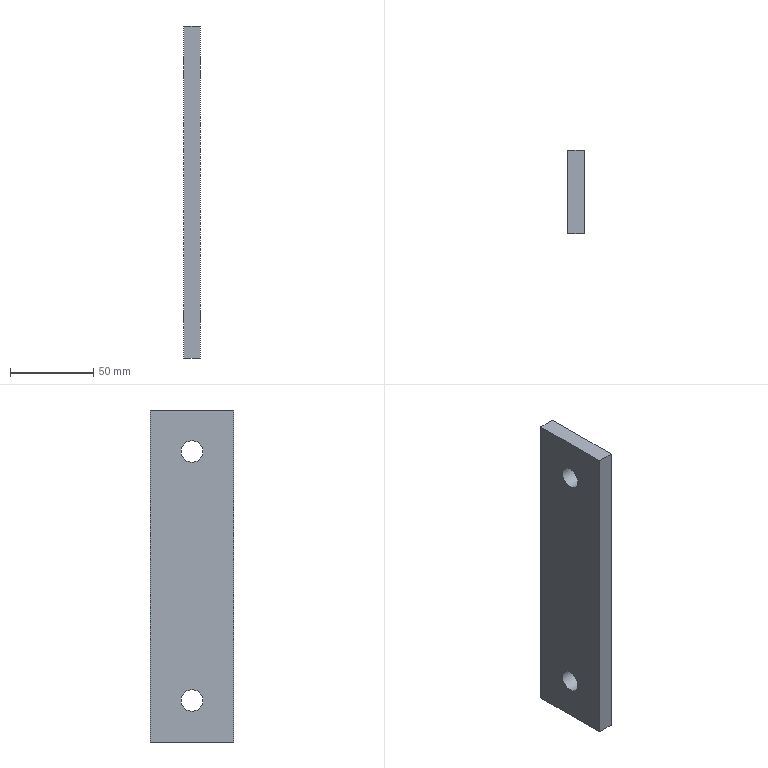Component | NX | BASE_FRAME_SHORT_CONN_PLATE | 1 solid | 8 faces | box 10 x 50 x 200 mm | volume 97345 mm3 | plane 6 | cylinder 2 | commonest cylinder face diameters 13 x2
STEP:
#1=CARTESIAN_POINT('',(0.,0.,0.));
#2=DIRECTION('',(0.,0.,1.));
#3=DIRECTION('',(1.,0.,0.));
#4=AXIS2_PLACEMENT_3D('',#1,#2,#3);
#5=CARTESIAN_POINT('',(-1250.,-50.,100.));
#6=VERTEX_POINT('',#5);
#7=CARTESIAN_POINT('',(-1250.,-50.,-100.));
#8=VERTEX_POINT('',#7);
#9=CARTESIAN_POINT('',(-1250.,-50.,100.));
#10=DIRECTION('',(0.,0.,-1.));
#11=VECTOR('',#10,1.);
#12=LINE('',#9,#11);
#13=CARTESIAN_POINT('',(-1260.,-50.,100.));
#14=DIRECTION('',(0.,-1.,0.));
#15=DIRECTION('',(1.,0.,0.));
#16=AXIS2_PLACEMENT_3D('',#13,#14,#15);
#17=PLANE('',#16);
#18=CARTESIAN_POINT('',(10.,0.));
#19=DIRECTION('',(0.,-1.));
#20=VECTOR('',#19,1.);
#21=LINE('',#18,#20);
#22=(GEOMETRIC_REPRESENTATION_CONTEXT(2)PARAMETRIC_REPRESENTATION_CONTEXT()REPRESENTATION_CONTEXT('',''));
#23=DEFINITIONAL_REPRESENTATION('',(#21),#22);
#24=PCURVE('',#17,#23);
#25=CARTESIAN_POINT('',(-1250.,-25.,75.));
#26=DIRECTION('',(-1.,0.,0.));
#27=DIRECTION('',(0.,0.,1.));
#28=AXIS2_PLACEMENT_3D('',#25,#26,#27);
#29=PLANE('',#28);
#30=CARTESIAN_POINT('',(25.,-25.));
#31=DIRECTION('',(-1.,0.));
#32=VECTOR('',#31,1.);
#33=LINE('',#30,#32);
#34=(GEOMETRIC_REPRESENTATION_CONTEXT(2)PARAMETRIC_REPRESENTATION_CONTEXT()REPRESENTATION_CONTEXT('',''));
#35=DEFINITIONAL_REPRESENTATION('',(#33),#34);
#36=PCURVE('',#29,#35);
#37=SURFACE_CURVE('',#12,(#24,#36),.PCURVE_S1.);
#38=EDGE_CURVE('',#6,#8,#37,.T.);
#39=ORIENTED_EDGE('',*,*,#38,.F.);
#40=CARTESIAN_POINT('',(-1260.,-50.,100.));
#41=VERTEX_POINT('',#40);
#42=CARTESIAN_POINT('',(-1260.,-50.,100.));
#43=DIRECTION('',(1.,0.,0.));
#44=VECTOR('',#43,1.);
#45=LINE('',#42,#44);
#46=CARTESIAN_POINT('',(0.,0.));
#47=DIRECTION('',(1.,0.));
#48=VECTOR('',#47,1.);
#49=LINE('',#46,#48);
#50=(GEOMETRIC_REPRESENTATION_CONTEXT(2)PARAMETRIC_REPRESENTATION_CONTEXT()REPRESENTATION_CONTEXT('',''));
#51=DEFINITIONAL_REPRESENTATION('',(#49),#50);
#52=PCURVE('',#17,#51);
#53=CARTESIAN_POINT('',(-1260.,0.,100.));
#54=DIRECTION('',(0.,0.,1.));
#55=DIRECTION('',(1.,0.,0.));
#56=AXIS2_PLACEMENT_3D('',#53,#54,#55);
#57=PLANE('',#56);
#58=CARTESIAN_POINT('',(0.,-50.));
#59=DIRECTION('',(1.,0.));
#60=VECTOR('',#59,1.);
#61=LINE('',#58,#60);
#62=(GEOMETRIC_REPRESENTATION_CONTEXT(2)PARAMETRIC_REPRESENTATION_CONTEXT()REPRESENTATION_CONTEXT('',''));
#63=DEFINITIONAL_REPRESENTATION('',(#61),#62);
#64=PCURVE('',#57,#63);
#65=SURFACE_CURVE('',#45,(#52,#64),.PCURVE_S1.);
#66=EDGE_CURVE('',#41,#6,#65,.T.);
#67=ORIENTED_EDGE('',*,*,#66,.F.);
#68=CARTESIAN_POINT('',(-1260.,-50.,-100.));
#69=VERTEX_POINT('',#68);
#70=CARTESIAN_POINT('',(-1260.,-50.,100.));
#71=DIRECTION('',(0.,0.,-1.));
#72=VECTOR('',#71,1.);
#73=LINE('',#70,#72);
#74=CARTESIAN_POINT('',(0.,0.));
#75=DIRECTION('',(0.,-1.));
#76=VECTOR('',#75,1.);
#77=LINE('',#74,#76);
#78=(GEOMETRIC_REPRESENTATION_CONTEXT(2)PARAMETRIC_REPRESENTATION_CONTEXT()REPRESENTATION_CONTEXT('',''));
#79=DEFINITIONAL_REPRESENTATION('',(#77),#78);
#80=PCURVE('',#17,#79);
#81=CARTESIAN_POINT('',(-1260.,-25.,75.));
#82=DIRECTION('',(-1.,0.,0.));
#83=DIRECTION('',(0.,0.,1.));
#84=AXIS2_PLACEMENT_3D('',#81,#82,#83);
#85=PLANE('',#84);
#86=CARTESIAN_POINT('',(25.,-25.));
#87=DIRECTION('',(-1.,0.));
#88=VECTOR('',#87,1.);
#89=LINE('',#86,#88);
#90=(GEOMETRIC_REPRESENTATION_CONTEXT(2)PARAMETRIC_REPRESENTATION_CONTEXT()REPRESENTATION_CONTEXT('',''));
#91=DEFINITIONAL_REPRESENTATION('',(#89),#90);
#92=PCURVE('',#85,#91);
#93=SURFACE_CURVE('',#73,(#80,#92),.PCURVE_S1.);
#94=EDGE_CURVE('',#41,#69,#93,.T.);
#95=ORIENTED_EDGE('',*,*,#94,.T.);
#96=CARTESIAN_POINT('',(-1260.,-50.,-100.));
#97=DIRECTION('',(1.,0.,0.));
#98=VECTOR('',#97,1.);
#99=LINE('',#96,#98);
#100=CARTESIAN_POINT('',(0.,-200.));
#101=DIRECTION('',(1.,0.));
#102=VECTOR('',#101,1.);
#103=LINE('',#100,#102);
#104=(GEOMETRIC_REPRESENTATION_CONTEXT(2)PARAMETRIC_REPRESENTATION_CONTEXT()REPRESENTATION_CONTEXT('',''));
#105=DEFINITIONAL_REPRESENTATION('',(#103),#104);
#106=PCURVE('',#17,#105);
#107=CARTESIAN_POINT('',(-1260.,-50.,-100.));
#108=DIRECTION('',(0.,0.,-1.));
#109=DIRECTION('',(-1.,0.,0.));
#110=AXIS2_PLACEMENT_3D('',#107,#108,#109);
#111=PLANE('',#110);
#112=CARTESIAN_POINT('',(0.,0.));
#113=DIRECTION('',(-1.,0.));
#114=VECTOR('',#113,1.);
#115=LINE('',#112,#114);
#116=(GEOMETRIC_REPRESENTATION_CONTEXT(2)PARAMETRIC_REPRESENTATION_CONTEXT()REPRESENTATION_CONTEXT('',''));
#117=DEFINITIONAL_REPRESENTATION('',(#115),#116);
#118=PCURVE('',#111,#117);
#119=SURFACE_CURVE('',#99,(#106,#118),.PCURVE_S1.);
#120=EDGE_CURVE('',#69,#8,#119,.T.);
#121=ORIENTED_EDGE('',*,*,#120,.T.);
#122=EDGE_LOOP('',(#39,#67,#95,#121));
#123=FACE_BOUND('',#122,.T.);
#124=ADVANCED_FACE('',(#123),#17,.T.);
#125=CARTESIAN_POINT('',(-1250.,0.,-100.));
#126=VERTEX_POINT('',#125);
#127=CARTESIAN_POINT('',(-1250.,-50.,-100.));
#128=DIRECTION('',(0.,1.,0.));
#129=VECTOR('',#128,1.);
#130=LINE('',#127,#129);
#131=CARTESIAN_POINT('',(-10.,0.));
#132=DIRECTION('',(0.,1.));
#133=VECTOR('',#132,1.);
#134=LINE('',#131,#133);
#135=(GEOMETRIC_REPRESENTATION_CONTEXT(2)PARAMETRIC_REPRESENTATION_CONTEXT()REPRESENTATION_CONTEXT('',''));
#136=DEFINITIONAL_REPRESENTATION('',(#134),#135);
#137=PCURVE('',#111,#136);
#138=CARTESIAN_POINT('',(-175.,-25.));
#139=DIRECTION('',(0.,1.));
#140=VECTOR('',#139,1.);
#141=LINE('',#138,#140);
#142=(GEOMETRIC_REPRESENTATION_CONTEXT(2)PARAMETRIC_REPRESENTATION_CONTEXT()REPRESENTATION_CONTEXT('',''));
#143=DEFINITIONAL_REPRESENTATION('',(#141),#142);
#144=PCURVE('',#29,#143);
#145=SURFACE_CURVE('',#130,(#137,#144),.PCURVE_S1.);
#146=EDGE_CURVE('',#8,#126,#145,.T.);
#147=ORIENTED_EDGE('',*,*,#146,.F.);
#148=ORIENTED_EDGE('',*,*,#120,.F.);
#149=CARTESIAN_POINT('',(-1260.,0.,-100.));
#150=VERTEX_POINT('',#149);
#151=CARTESIAN_POINT('',(-1260.,-50.,-100.));
#152=DIRECTION('',(0.,1.,0.));
#153=VECTOR('',#152,1.);
#154=LINE('',#151,#153);
#155=CARTESIAN_POINT('',(0.,0.));
#156=DIRECTION('',(0.,1.));
#157=VECTOR('',#156,1.);
#158=LINE('',#155,#157);
#159=(GEOMETRIC_REPRESENTATION_CONTEXT(2)PARAMETRIC_REPRESENTATION_CONTEXT()REPRESENTATION_CONTEXT('',''));
#160=DEFINITIONAL_REPRESENTATION('',(#158),#159);
#161=PCURVE('',#111,#160);
#162=CARTESIAN_POINT('',(-175.,-25.));
#163=DIRECTION('',(0.,1.));
#164=VECTOR('',#163,1.);
#165=LINE('',#162,#164);
#166=(GEOMETRIC_REPRESENTATION_CONTEXT(2)PARAMETRIC_REPRESENTATION_CONTEXT()REPRESENTATION_CONTEXT('',''));
#167=DEFINITIONAL_REPRESENTATION('',(#165),#166);
#168=PCURVE('',#85,#167);
#169=SURFACE_CURVE('',#154,(#161,#168),.PCURVE_S1.);
#170=EDGE_CURVE('',#69,#150,#169,.T.);
#171=ORIENTED_EDGE('',*,*,#170,.T.);
#172=CARTESIAN_POINT('',(-1260.,0.,-100.));
#173=DIRECTION('',(1.,0.,0.));
#174=VECTOR('',#173,1.);
#175=LINE('',#172,#174);
#176=CARTESIAN_POINT('',(0.,50.));
#177=DIRECTION('',(-1.,0.));
#178=VECTOR('',#177,1.);
#179=LINE('',#176,#178);
#180=(GEOMETRIC_REPRESENTATION_CONTEXT(2)PARAMETRIC_REPRESENTATION_CONTEXT()REPRESENTATION_CONTEXT('',''));
#181=DEFINITIONAL_REPRESENTATION('',(#179),#180);
#182=PCURVE('',#111,#181);
#183=CARTESIAN_POINT('',(-1260.,0.,-100.));
#184=DIRECTION('',(0.,1.,0.));
#185=DIRECTION('',(-1.,0.,0.));
#186=AXIS2_PLACEMENT_3D('',#183,#184,#185);
#187=PLANE('',#186);
#188=CARTESIAN_POINT('',(0.,0.));
#189=DIRECTION('',(-1.,0.));
#190=VECTOR('',#189,1.);
#191=LINE('',#188,#190);
#192=(GEOMETRIC_REPRESENTATION_CONTEXT(2)PARAMETRIC_REPRESENTATION_CONTEXT()REPRESENTATION_CONTEXT('',''));
#193=DEFINITIONAL_REPRESENTATION('',(#191),#192);
#194=PCURVE('',#187,#193);
#195=SURFACE_CURVE('',#175,(#182,#194),.PCURVE_S1.);
#196=EDGE_CURVE('',#150,#126,#195,.T.);
#197=ORIENTED_EDGE('',*,*,#196,.T.);
#198=EDGE_LOOP('',(#147,#148,#171,#197));
#199=FACE_BOUND('',#198,.T.);
#200=ADVANCED_FACE('',(#199),#111,.T.);
#201=CARTESIAN_POINT('',(-1250.,0.,100.));
#202=VERTEX_POINT('',#201);
#203=CARTESIAN_POINT('',(-1250.,0.,-100.));
#204=DIRECTION('',(0.,0.,1.));
#205=VECTOR('',#204,1.);
#206=LINE('',#203,#205);
#207=CARTESIAN_POINT('',(-10.,0.));
#208=DIRECTION('',(0.,1.));
#209=VECTOR('',#208,1.);
#210=LINE('',#207,#209);
#211=(GEOMETRIC_REPRESENTATION_CONTEXT(2)PARAMETRIC_REPRESENTATION_CONTEXT()REPRESENTATION_CONTEXT('',''));
#212=DEFINITIONAL_REPRESENTATION('',(#210),#211);
#213=PCURVE('',#187,#212);
#214=CARTESIAN_POINT('',(-175.,25.));
#215=DIRECTION('',(1.,0.));
#216=VECTOR('',#215,1.);
#217=LINE('',#214,#216);
#218=(GEOMETRIC_REPRESENTATION_CONTEXT(2)PARAMETRIC_REPRESENTATION_CONTEXT()REPRESENTATION_CONTEXT('',''));
#219=DEFINITIONAL_REPRESENTATION('',(#217),#218);
#220=PCURVE('',#29,#219);
#221=SURFACE_CURVE('',#206,(#213,#220),.PCURVE_S1.);
#222=EDGE_CURVE('',#126,#202,#221,.T.);
#223=ORIENTED_EDGE('',*,*,#222,.F.);
#224=ORIENTED_EDGE('',*,*,#196,.F.);
#225=CARTESIAN_POINT('',(-1260.,0.,100.));
#226=VERTEX_POINT('',#225);
#227=CARTESIAN_POINT('',(-1260.,0.,-100.));
#228=DIRECTION('',(0.,0.,1.));
#229=VECTOR('',#228,1.);
#230=LINE('',#227,#229);
#231=CARTESIAN_POINT('',(0.,0.));
#232=DIRECTION('',(0.,1.));
#233=VECTOR('',#232,1.);
#234=LINE('',#231,#233);
#235=(GEOMETRIC_REPRESENTATION_CONTEXT(2)PARAMETRIC_REPRESENTATION_CONTEXT()REPRESENTATION_CONTEXT('',''));
#236=DEFINITIONAL_REPRESENTATION('',(#234),#235);
#237=PCURVE('',#187,#236);
#238=CARTESIAN_POINT('',(-175.,25.));
#239=DIRECTION('',(1.,0.));
#240=VECTOR('',#239,1.);
#241=LINE('',#238,#240);
#242=(GEOMETRIC_REPRESENTATION_CONTEXT(2)PARAMETRIC_REPRESENTATION_CONTEXT()REPRESENTATION_CONTEXT('',''));
#243=DEFINITIONAL_REPRESENTATION('',(#241),#242);
#244=PCURVE('',#85,#243);
#245=SURFACE_CURVE('',#230,(#237,#244),.PCURVE_S1.);
#246=EDGE_CURVE('',#150,#226,#245,.T.);
#247=ORIENTED_EDGE('',*,*,#246,.T.);
#248=CARTESIAN_POINT('',(-1260.,0.,100.));
#249=DIRECTION('',(1.,0.,0.));
#250=VECTOR('',#249,1.);
#251=LINE('',#248,#250);
#252=CARTESIAN_POINT('',(0.,200.));
#253=DIRECTION('',(-1.,0.));
#254=VECTOR('',#253,1.);
#255=LINE('',#252,#254);
#256=(GEOMETRIC_REPRESENTATION_CONTEXT(2)PARAMETRIC_REPRESENTATION_CONTEXT()REPRESENTATION_CONTEXT('',''));
#257=DEFINITIONAL_REPRESENTATION('',(#255),#256);
#258=PCURVE('',#187,#257);
#259=CARTESIAN_POINT('',(0.,0.));
#260=DIRECTION('',(1.,0.));
#261=VECTOR('',#260,1.);
#262=LINE('',#259,#261);
#263=(GEOMETRIC_REPRESENTATION_CONTEXT(2)PARAMETRIC_REPRESENTATION_CONTEXT()REPRESENTATION_CONTEXT('',''));
#264=DEFINITIONAL_REPRESENTATION('',(#262),#263);
#265=PCURVE('',#57,#264);
#266=SURFACE_CURVE('',#251,(#258,#265),.PCURVE_S1.);
#267=EDGE_CURVE('',#226,#202,#266,.T.);
#268=ORIENTED_EDGE('',*,*,#267,.T.);
#269=EDGE_LOOP('',(#223,#224,#247,#268));
#270=FACE_BOUND('',#269,.T.);
#271=ADVANCED_FACE('',(#270),#187,.T.);
#272=CARTESIAN_POINT('',(-1260.,-25.,68.5));
#273=VERTEX_POINT('',#272);
#274=CARTESIAN_POINT('',(-1260.,-25.,75.));
#275=DIRECTION('',(-1.,0.,0.));
#276=DIRECTION('',(0.,0.,-1.));
#277=AXIS2_PLACEMENT_3D('',#274,#275,#276);
#278=CIRCLE('',#277,6.5);
#279=CARTESIAN_POINT('',(-1260.,-25.,75.));
#280=DIRECTION('',(1.,0.,0.));
#281=DIRECTION('',(0.,0.,-1.));
#282=AXIS2_PLACEMENT_3D('',#279,#280,#281);
#283=CYLINDRICAL_SURFACE('',#282,6.5);
#284=CARTESIAN_POINT('',(6.283,0.));
#285=DIRECTION('',(-1.,0.));
#286=VECTOR('',#285,1.);
#287=LINE('',#284,#286);
#288=(GEOMETRIC_REPRESENTATION_CONTEXT(2)PARAMETRIC_REPRESENTATION_CONTEXT()REPRESENTATION_CONTEXT('',''));
#289=DEFINITIONAL_REPRESENTATION('',(#287),#288);
#290=PCURVE('',#283,#289);
#291=CARTESIAN_POINT('',(0.,0.));
#292=DIRECTION('',(-1.,0.));
#293=AXIS2_PLACEMENT_2D('',#291,#292);
#294=CIRCLE('',#293,6.5);
#295=(GEOMETRIC_REPRESENTATION_CONTEXT(2)PARAMETRIC_REPRESENTATION_CONTEXT()REPRESENTATION_CONTEXT('',''));
#296=DEFINITIONAL_REPRESENTATION('',(#294),#295);
#297=PCURVE('',#85,#296);
#298=SURFACE_CURVE('',#278,(#290,#297),.PCURVE_S1.);
#299=EDGE_CURVE('',#273,#273,#298,.T.);
#300=ORIENTED_EDGE('',*,*,#299,.F.);
#301=CARTESIAN_POINT('',(-1250.,-25.,68.5));
#302=VERTEX_POINT('',#301);
#303=CARTESIAN_POINT('',(-1260.,-25.,68.5));
#304=CARTESIAN_POINT('',(-1250.,-25.,68.5));
#305=B_SPLINE_CURVE_WITH_KNOTS('',1,(#303,#304),.UNSPECIFIED.,.F.,.F.,(2,2),(0.,10.),.PIECEWISE_BEZIER_KNOTS.);
#306=CARTESIAN_POINT('',(6.283,0.));
#307=DIRECTION('',(0.,1.));
#308=VECTOR('',#307,1.);
#309=LINE('',#306,#308);
#310=(GEOMETRIC_REPRESENTATION_CONTEXT(2)PARAMETRIC_REPRESENTATION_CONTEXT()REPRESENTATION_CONTEXT('',''));
#311=DEFINITIONAL_REPRESENTATION('',(#309),#310);
#312=PCURVE('',#283,#311);
#313=CARTESIAN_POINT('',(0.,0.));
#314=DIRECTION('',(0.,1.));
#315=VECTOR('',#314,1.);
#316=LINE('',#313,#315);
#317=(GEOMETRIC_REPRESENTATION_CONTEXT(2)PARAMETRIC_REPRESENTATION_CONTEXT()REPRESENTATION_CONTEXT('',''));
#318=DEFINITIONAL_REPRESENTATION('',(#316),#317);
#319=PCURVE('',#283,#318);
#320=SEAM_CURVE('',#305,(#312,#319),.PCURVE_S1.);
#321=EDGE_CURVE('',#273,#302,#320,.T.);
#322=ORIENTED_EDGE('',*,*,#321,.T.);
#323=CARTESIAN_POINT('',(-1250.,-25.,75.));
#324=DIRECTION('',(-1.,0.,0.));
#325=DIRECTION('',(0.,0.,-1.));
#326=AXIS2_PLACEMENT_3D('',#323,#324,#325);
#327=CIRCLE('',#326,6.5);
#328=CARTESIAN_POINT('',(6.283,10.));
#329=DIRECTION('',(-1.,0.));
#330=VECTOR('',#329,1.);
#331=LINE('',#328,#330);
#332=(GEOMETRIC_REPRESENTATION_CONTEXT(2)PARAMETRIC_REPRESENTATION_CONTEXT()REPRESENTATION_CONTEXT('',''));
#333=DEFINITIONAL_REPRESENTATION('',(#331),#332);
#334=PCURVE('',#283,#333);
#335=CARTESIAN_POINT('',(0.,0.));
#336=DIRECTION('',(-1.,0.));
#337=AXIS2_PLACEMENT_2D('',#335,#336);
#338=CIRCLE('',#337,6.5);
#339=(GEOMETRIC_REPRESENTATION_CONTEXT(2)PARAMETRIC_REPRESENTATION_CONTEXT()REPRESENTATION_CONTEXT('',''));
#340=DEFINITIONAL_REPRESENTATION('',(#338),#339);
#341=PCURVE('',#29,#340);
#342=SURFACE_CURVE('',#327,(#334,#341),.PCURVE_S1.);
#343=EDGE_CURVE('',#302,#302,#342,.T.);
#344=ORIENTED_EDGE('',*,*,#343,.T.);
#345=ORIENTED_EDGE('',*,*,#321,.F.);
#346=EDGE_LOOP('',(#300,#322,#344,#345));
#347=FACE_BOUND('',#346,.F.);
#348=ADVANCED_FACE('',(#347),#283,.F.);
#349=CARTESIAN_POINT('',(-1250.,0.,100.));
#350=DIRECTION('',(0.,-1.,0.));
#351=VECTOR('',#350,1.);
#352=LINE('',#349,#351);
#353=CARTESIAN_POINT('',(10.,0.));
#354=DIRECTION('',(0.,-1.));
#355=VECTOR('',#354,1.);
#356=LINE('',#353,#355);
#357=(GEOMETRIC_REPRESENTATION_CONTEXT(2)PARAMETRIC_REPRESENTATION_CONTEXT()REPRESENTATION_CONTEXT('',''));
#358=DEFINITIONAL_REPRESENTATION('',(#356),#357);
#359=PCURVE('',#57,#358);
#360=CARTESIAN_POINT('',(25.,25.));
#361=DIRECTION('',(0.,-1.));
#362=VECTOR('',#361,1.);
#363=LINE('',#360,#362);
#364=(GEOMETRIC_REPRESENTATION_CONTEXT(2)PARAMETRIC_REPRESENTATION_CONTEXT()REPRESENTATION_CONTEXT('',''));
#365=DEFINITIONAL_REPRESENTATION('',(#363),#364);
#366=PCURVE('',#29,#365);
#367=SURFACE_CURVE('',#352,(#359,#366),.PCURVE_S1.);
#368=EDGE_CURVE('',#202,#6,#367,.T.);
#369=ORIENTED_EDGE('',*,*,#368,.F.);
#370=ORIENTED_EDGE('',*,*,#267,.F.);
#371=CARTESIAN_POINT('',(-1260.,0.,100.));
#372=DIRECTION('',(0.,-1.,0.));
#373=VECTOR('',#372,1.);
#374=LINE('',#371,#373);
#375=CARTESIAN_POINT('',(0.,0.));
#376=DIRECTION('',(0.,-1.));
#377=VECTOR('',#376,1.);
#378=LINE('',#375,#377);
#379=(GEOMETRIC_REPRESENTATION_CONTEXT(2)PARAMETRIC_REPRESENTATION_CONTEXT()REPRESENTATION_CONTEXT('',''));
#380=DEFINITIONAL_REPRESENTATION('',(#378),#379);
#381=PCURVE('',#57,#380);
#382=CARTESIAN_POINT('',(25.,25.));
#383=DIRECTION('',(0.,-1.));
#384=VECTOR('',#383,1.);
#385=LINE('',#382,#384);
#386=(GEOMETRIC_REPRESENTATION_CONTEXT(2)PARAMETRIC_REPRESENTATION_CONTEXT()REPRESENTATION_CONTEXT('',''));
#387=DEFINITIONAL_REPRESENTATION('',(#385),#386);
#388=PCURVE('',#85,#387);
#389=SURFACE_CURVE('',#374,(#381,#388),.PCURVE_S1.);
#390=EDGE_CURVE('',#226,#41,#389,.T.);
#391=ORIENTED_EDGE('',*,*,#390,.T.);
#392=ORIENTED_EDGE('',*,*,#66,.T.);
#393=EDGE_LOOP('',(#369,#370,#391,#392));
#394=FACE_BOUND('',#393,.T.);
#395=ADVANCED_FACE('',(#394),#57,.T.);
#396=CARTESIAN_POINT('',(-1260.,-25.,-68.5));
#397=VERTEX_POINT('',#396);
#398=CARTESIAN_POINT('',(-1260.,-25.,-75.));
#399=DIRECTION('',(1.,0.,0.));
#400=DIRECTION('',(0.,0.,1.));
#401=AXIS2_PLACEMENT_3D('',#398,#399,#400);
#402=CIRCLE('',#401,6.5);
#403=CARTESIAN_POINT('',(-1260.,-25.,-75.));
#404=DIRECTION('',(1.,0.,0.));
#405=DIRECTION('',(0.,0.,-1.));
#406=AXIS2_PLACEMENT_3D('',#403,#404,#405);
#407=CYLINDRICAL_SURFACE('',#406,6.5);
#408=CARTESIAN_POINT('',(3.142,0.));
#409=DIRECTION('',(1.,0.));
#410=VECTOR('',#409,1.);
#411=LINE('',#408,#410);
#412=(GEOMETRIC_REPRESENTATION_CONTEXT(2)PARAMETRIC_REPRESENTATION_CONTEXT()REPRESENTATION_CONTEXT('',''));
#413=DEFINITIONAL_REPRESENTATION('',(#411),#412);
#414=PCURVE('',#407,#413);
#415=CARTESIAN_POINT('',(-143.5,0.));
#416=CARTESIAN_POINT('',(-143.5,-11.258));
#417=CARTESIAN_POINT('',(-153.25,-5.629));
#418=CARTESIAN_POINT('',(-163.,-0.));
#419=CARTESIAN_POINT('',(-153.25,5.629));
#420=CARTESIAN_POINT('',(-143.5,11.258));
#421=CARTESIAN_POINT('',(-143.5,0.));
#422=(BOUNDED_CURVE()B_SPLINE_CURVE(2,(#415,#416,#417,#418,#419,#420,#421),.UNSPECIFIED.,.T.,.F.)B_SPLINE_CURVE_WITH_KNOTS((1,2,2,2,2,1),(-2.094,0.,2.094,4.189,6.283,8.378),.UNSPECIFIED.)CURVE()GEOMETRIC_REPRESENTATION_ITEM()RATIONAL_B_SPLINE_CURVE((1.,0.5,1.,0.5,1.,0.5,1.))REPRESENTATION_ITEM(''));
#423=(GEOMETRIC_REPRESENTATION_CONTEXT(2)PARAMETRIC_REPRESENTATION_CONTEXT()REPRESENTATION_CONTEXT('',''));
#424=DEFINITIONAL_REPRESENTATION('',(#422),#423);
#425=PCURVE('',#85,#424);
#426=SURFACE_CURVE('',#402,(#414,#425),.PCURVE_S1.);
#427=EDGE_CURVE('',#397,#397,#426,.T.);
#428=ORIENTED_EDGE('',*,*,#427,.T.);
#429=CARTESIAN_POINT('',(-1250.,-25.,-68.5));
#430=VERTEX_POINT('',#429);
#431=CARTESIAN_POINT('',(-1260.,-25.,-68.5));
#432=CARTESIAN_POINT('',(-1250.,-25.,-68.5));
#433=B_SPLINE_CURVE_WITH_KNOTS('',1,(#431,#432),.UNSPECIFIED.,.F.,.F.,(2,2),(0.,10.),.PIECEWISE_BEZIER_KNOTS.);
#434=CARTESIAN_POINT('',(9.425,0.));
#435=DIRECTION('',(0.,1.));
#436=VECTOR('',#435,1.);
#437=LINE('',#434,#436);
#438=(GEOMETRIC_REPRESENTATION_CONTEXT(2)PARAMETRIC_REPRESENTATION_CONTEXT()REPRESENTATION_CONTEXT('',''));
#439=DEFINITIONAL_REPRESENTATION('',(#437),#438);
#440=PCURVE('',#407,#439);
#441=CARTESIAN_POINT('',(3.142,0.));
#442=DIRECTION('',(0.,1.));
#443=VECTOR('',#442,1.);
#444=LINE('',#441,#443);
#445=(GEOMETRIC_REPRESENTATION_CONTEXT(2)PARAMETRIC_REPRESENTATION_CONTEXT()REPRESENTATION_CONTEXT('',''));
#446=DEFINITIONAL_REPRESENTATION('',(#444),#445);
#447=PCURVE('',#407,#446);
#448=SEAM_CURVE('',#433,(#440,#447),.PCURVE_S1.);
#449=EDGE_CURVE('',#397,#430,#448,.T.);
#450=ORIENTED_EDGE('',*,*,#449,.T.);
#451=CARTESIAN_POINT('',(-1250.,-25.,-75.));
#452=DIRECTION('',(1.,0.,0.));
#453=DIRECTION('',(0.,0.,1.));
#454=AXIS2_PLACEMENT_3D('',#451,#452,#453);
#455=CIRCLE('',#454,6.5);
#456=CARTESIAN_POINT('',(3.142,10.));
#457=DIRECTION('',(1.,0.));
#458=VECTOR('',#457,1.);
#459=LINE('',#456,#458);
#460=(GEOMETRIC_REPRESENTATION_CONTEXT(2)PARAMETRIC_REPRESENTATION_CONTEXT()REPRESENTATION_CONTEXT('',''));
#461=DEFINITIONAL_REPRESENTATION('',(#459),#460);
#462=PCURVE('',#407,#461);
#463=CARTESIAN_POINT('',(-143.5,0.));
#464=CARTESIAN_POINT('',(-143.5,-11.258));
#465=CARTESIAN_POINT('',(-153.25,-5.629));
#466=CARTESIAN_POINT('',(-163.,-0.));
#467=CARTESIAN_POINT('',(-153.25,5.629));
#468=CARTESIAN_POINT('',(-143.5,11.258));
#469=CARTESIAN_POINT('',(-143.5,0.));
#470=(BOUNDED_CURVE()B_SPLINE_CURVE(2,(#463,#464,#465,#466,#467,#468,#469),.UNSPECIFIED.,.T.,.F.)B_SPLINE_CURVE_WITH_KNOTS((1,2,2,2,2,1),(-2.094,0.,2.094,4.189,6.283,8.378),.UNSPECIFIED.)CURVE()GEOMETRIC_REPRESENTATION_ITEM()RATIONAL_B_SPLINE_CURVE((1.,0.5,1.,0.5,1.,0.5,1.))REPRESENTATION_ITEM(''));
#471=(GEOMETRIC_REPRESENTATION_CONTEXT(2)PARAMETRIC_REPRESENTATION_CONTEXT()REPRESENTATION_CONTEXT('',''));
#472=DEFINITIONAL_REPRESENTATION('',(#470),#471);
#473=PCURVE('',#29,#472);
#474=SURFACE_CURVE('',#455,(#462,#473),.PCURVE_S1.);
#475=EDGE_CURVE('',#430,#430,#474,.T.);
#476=ORIENTED_EDGE('',*,*,#475,.F.);
#477=ORIENTED_EDGE('',*,*,#449,.F.);
#478=EDGE_LOOP('',(#428,#450,#476,#477));
#479=FACE_BOUND('',#478,.F.);
#480=ADVANCED_FACE('',(#479),#407,.F.);
#481=ORIENTED_EDGE('',*,*,#94,.F.);
#482=ORIENTED_EDGE('',*,*,#390,.F.);
#483=ORIENTED_EDGE('',*,*,#246,.F.);
#484=ORIENTED_EDGE('',*,*,#170,.F.);
#485=EDGE_LOOP('',(#481,#482,#483,#484));
#486=FACE_BOUND('',#485,.T.);
#487=ORIENTED_EDGE('',*,*,#299,.F.);
#488=EDGE_LOOP('',(#487));
#489=FACE_BOUND('',#488,.T.);
#490=ORIENTED_EDGE('',*,*,#427,.T.);
#491=EDGE_LOOP('',(#490));
#492=FACE_BOUND('',#491,.T.);
#493=ADVANCED_FACE('',(#486,#489,#492),#85,.T.);
#494=ORIENTED_EDGE('',*,*,#38,.T.);
#495=ORIENTED_EDGE('',*,*,#146,.T.);
#496=ORIENTED_EDGE('',*,*,#222,.T.);
#497=ORIENTED_EDGE('',*,*,#368,.T.);
#498=EDGE_LOOP('',(#494,#495,#496,#497));
#499=FACE_BOUND('',#498,.T.);
#500=ORIENTED_EDGE('',*,*,#343,.T.);
#501=EDGE_LOOP('',(#500));
#502=FACE_BOUND('',#501,.T.);
#503=ORIENTED_EDGE('',*,*,#475,.F.);
#504=EDGE_LOOP('',(#503));
#505=FACE_BOUND('',#504,.T.);
#506=ADVANCED_FACE('',(#499,#502,#505),#29,.F.);
#507=CLOSED_SHELL('',(#124,#200,#271,#348,#395,#480,#493,#506));
#508=MANIFOLD_SOLID_BREP('',#507);
#509=(LENGTH_UNIT()NAMED_UNIT(*)SI_UNIT(.MILLI.,.METRE.));
#510=UNCERTAINTY_MEASURE_WITH_UNIT(LENGTH_MEASURE(0.000002),#509,'','');
#511=(NAMED_UNIT(*)PLANE_ANGLE_UNIT()SI_UNIT($,.RADIAN.));
#512=(NAMED_UNIT(*)SI_UNIT($,.STERADIAN.)SOLID_ANGLE_UNIT());
#513=(GEOMETRIC_REPRESENTATION_CONTEXT(3)GLOBAL_UNCERTAINTY_ASSIGNED_CONTEXT((#510))GLOBAL_UNIT_ASSIGNED_CONTEXT((#509,#511,#512))REPRESENTATION_CONTEXT('',''));
#514=ADVANCED_BREP_SHAPE_REPRESENTATION('',(#4,#508),#513);